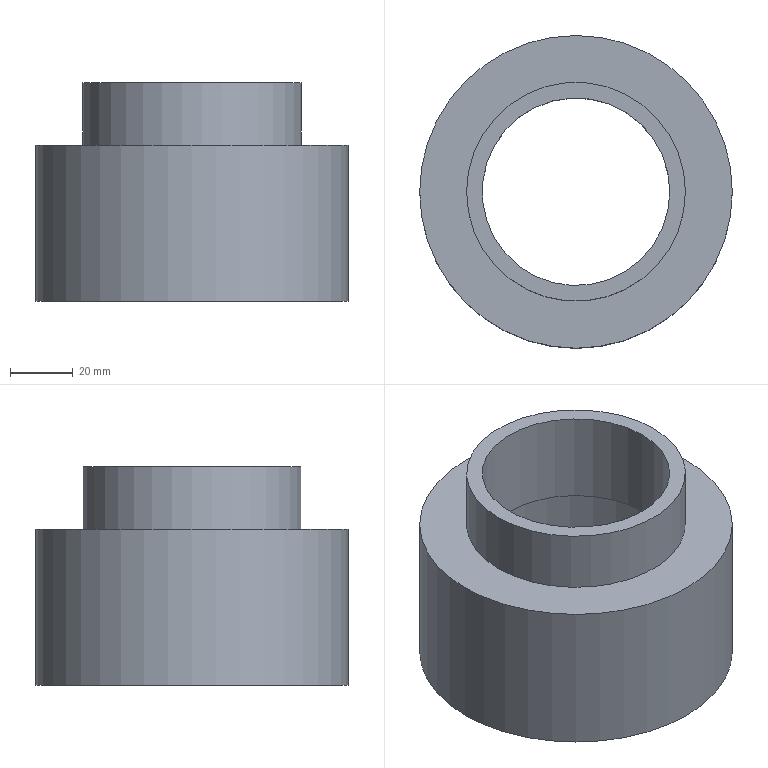Component | NX | CONNECTING_SLEEVE | 1 solid | 8 faces | box 100 x 100 x 70 mm | volume 130376 mm3 | plane 4 | cylinder 4 | commonest cylinder face diameters 100 x1 70 x1 60 x1 90 x1
STEP:
#1=CARTESIAN_POINT('',(0.,0.,0.));
#2=DIRECTION('',(0.,0.,1.));
#3=DIRECTION('',(1.,0.,0.));
#4=AXIS2_PLACEMENT_3D('',#1,#2,#3);
#5=CARTESIAN_POINT('',(35.,0.,-612.5));
#6=VERTEX_POINT('',#5);
#7=CARTESIAN_POINT('',(-0.,0.,-612.5));
#8=DIRECTION('',(0.,0.,1.));
#9=DIRECTION('',(1.,0.,0.));
#10=AXIS2_PLACEMENT_3D('',#7,#8,#9);
#11=CIRCLE('',#10,35.);
#12=CARTESIAN_POINT('',(0.,0.,-612.5));
#13=DIRECTION('',(0.,0.,1.));
#14=DIRECTION('',(1.,0.,0.));
#15=AXIS2_PLACEMENT_3D('',#12,#13,#14);
#16=PLANE('',#15);
#17=CARTESIAN_POINT('',(-0.,-0.));
#18=DIRECTION('',(1.,0.));
#19=AXIS2_PLACEMENT_2D('',#17,#18);
#20=CIRCLE('',#19,35.);
#21=(GEOMETRIC_REPRESENTATION_CONTEXT(2)PARAMETRIC_REPRESENTATION_CONTEXT()REPRESENTATION_CONTEXT('',''));
#22=DEFINITIONAL_REPRESENTATION('',(#20),#21);
#23=PCURVE('',#16,#22);
#24=CARTESIAN_POINT('',(-0.,0.,-612.5));
#25=DIRECTION('',(0.,0.,1.));
#26=DIRECTION('',(1.,0.,0.));
#27=AXIS2_PLACEMENT_3D('',#24,#25,#26);
#28=CYLINDRICAL_SURFACE('',#27,35.);
#29=CARTESIAN_POINT('',(0.,0.));
#30=DIRECTION('',(1.,0.));
#31=VECTOR('',#30,1.);
#32=LINE('',#29,#31);
#33=(GEOMETRIC_REPRESENTATION_CONTEXT(2)PARAMETRIC_REPRESENTATION_CONTEXT()REPRESENTATION_CONTEXT('',''));
#34=DEFINITIONAL_REPRESENTATION('',(#32),#33);
#35=PCURVE('',#28,#34);
#36=SURFACE_CURVE('',#11,(#23,#35),.PCURVE_S1.);
#37=EDGE_CURVE('',#6,#6,#36,.T.);
#38=ORIENTED_EDGE('',*,*,#37,.F.);
#39=EDGE_LOOP('',(#38));
#40=FACE_BOUND('',#39,.T.);
#41=CARTESIAN_POINT('',(50.,0.,-612.5));
#42=VERTEX_POINT('',#41);
#43=CARTESIAN_POINT('',(0.,0.,-612.5));
#44=DIRECTION('',(0.,0.,-1.));
#45=DIRECTION('',(1.,0.,0.));
#46=AXIS2_PLACEMENT_3D('',#43,#44,#45);
#47=CIRCLE('',#46,50.);
#48=CARTESIAN_POINT('',(50.,0.));
#49=CARTESIAN_POINT('',(50.,-86.603));
#50=CARTESIAN_POINT('',(-25.,-43.301));
#51=CARTESIAN_POINT('',(-100.,-0.));
#52=CARTESIAN_POINT('',(-25.,43.301));
#53=CARTESIAN_POINT('',(50.,86.603));
#54=CARTESIAN_POINT('',(50.,0.));
#55=(BOUNDED_CURVE()B_SPLINE_CURVE(2,(#48,#49,#50,#51,#52,#53,#54),.UNSPECIFIED.,.T.,.F.)B_SPLINE_CURVE_WITH_KNOTS((1,2,2,2,2,1),(-2.094,0.,2.094,4.189,6.283,8.378),.UNSPECIFIED.)CURVE()GEOMETRIC_REPRESENTATION_ITEM()RATIONAL_B_SPLINE_CURVE((1.,0.5,1.,0.5,1.,0.5,1.))REPRESENTATION_ITEM(''));
#56=(GEOMETRIC_REPRESENTATION_CONTEXT(2)PARAMETRIC_REPRESENTATION_CONTEXT()REPRESENTATION_CONTEXT('',''));
#57=DEFINITIONAL_REPRESENTATION('',(#55),#56);
#58=PCURVE('',#16,#57);
#59=CARTESIAN_POINT('',(0.,0.,-662.5));
#60=DIRECTION('',(0.,0.,1.));
#61=DIRECTION('',(1.,0.,0.));
#62=AXIS2_PLACEMENT_3D('',#59,#60,#61);
#63=CYLINDRICAL_SURFACE('',#62,50.);
#64=CARTESIAN_POINT('',(6.283,50.));
#65=DIRECTION('',(-1.,0.));
#66=VECTOR('',#65,1.);
#67=LINE('',#64,#66);
#68=(GEOMETRIC_REPRESENTATION_CONTEXT(2)PARAMETRIC_REPRESENTATION_CONTEXT()REPRESENTATION_CONTEXT('',''));
#69=DEFINITIONAL_REPRESENTATION('',(#67),#68);
#70=PCURVE('',#63,#69);
#71=SURFACE_CURVE('',#47,(#58,#70),.PCURVE_S1.);
#72=EDGE_CURVE('',#42,#42,#71,.T.);
#73=ORIENTED_EDGE('',*,*,#72,.F.);
#74=EDGE_LOOP('',(#73));
#75=FACE_BOUND('',#74,.T.);
#76=ADVANCED_FACE('',(#40,#75),#16,.T.);
#77=CARTESIAN_POINT('',(45.,0.,-662.5));
#78=VERTEX_POINT('',#77);
#79=CARTESIAN_POINT('',(-0.,0.,-662.5));
#80=DIRECTION('',(0.,0.,1.));
#81=DIRECTION('',(1.,0.,0.));
#82=AXIS2_PLACEMENT_3D('',#79,#80,#81);
#83=CIRCLE('',#82,45.);
#84=CARTESIAN_POINT('',(0.,0.,-662.5));
#85=DIRECTION('',(0.,0.,-1.));
#86=DIRECTION('',(-1.,0.,0.));
#87=AXIS2_PLACEMENT_3D('',#84,#85,#86);
#88=PLANE('',#87);
#89=CARTESIAN_POINT('',(-45.,-0.));
#90=CARTESIAN_POINT('',(-45.,77.942));
#91=CARTESIAN_POINT('',(22.5,38.971));
#92=CARTESIAN_POINT('',(90.,0.));
#93=CARTESIAN_POINT('',(22.5,-38.971));
#94=CARTESIAN_POINT('',(-45.,-77.942));
#95=CARTESIAN_POINT('',(-45.,-0.));
#96=(BOUNDED_CURVE()B_SPLINE_CURVE(2,(#89,#90,#91,#92,#93,#94,#95),.UNSPECIFIED.,.T.,.F.)B_SPLINE_CURVE_WITH_KNOTS((1,2,2,2,2,1),(-2.094,0.,2.094,4.189,6.283,8.378),.UNSPECIFIED.)CURVE()GEOMETRIC_REPRESENTATION_ITEM()RATIONAL_B_SPLINE_CURVE((1.,0.5,1.,0.5,1.,0.5,1.))REPRESENTATION_ITEM(''));
#97=(GEOMETRIC_REPRESENTATION_CONTEXT(2)PARAMETRIC_REPRESENTATION_CONTEXT()REPRESENTATION_CONTEXT('',''));
#98=DEFINITIONAL_REPRESENTATION('',(#96),#97);
#99=PCURVE('',#88,#98);
#100=CARTESIAN_POINT('',(-0.,0.,-622.5));
#101=DIRECTION('',(0.,0.,-1.));
#102=DIRECTION('',(-1.,0.,0.));
#103=AXIS2_PLACEMENT_3D('',#100,#101,#102);
#104=CYLINDRICAL_SURFACE('',#103,45.);
#105=CARTESIAN_POINT('',(9.425,40.));
#106=DIRECTION('',(-1.,0.));
#107=VECTOR('',#106,1.);
#108=LINE('',#105,#107);
#109=(GEOMETRIC_REPRESENTATION_CONTEXT(2)PARAMETRIC_REPRESENTATION_CONTEXT()REPRESENTATION_CONTEXT('',''));
#110=DEFINITIONAL_REPRESENTATION('',(#108),#109);
#111=PCURVE('',#104,#110);
#112=SURFACE_CURVE('',#83,(#99,#111),.PCURVE_S1.);
#113=EDGE_CURVE('',#78,#78,#112,.T.);
#114=ORIENTED_EDGE('',*,*,#113,.T.);
#115=EDGE_LOOP('',(#114));
#116=FACE_BOUND('',#115,.T.);
#117=CARTESIAN_POINT('',(50.,0.,-662.5));
#118=VERTEX_POINT('',#117);
#119=CARTESIAN_POINT('',(0.,0.,-662.5));
#120=DIRECTION('',(0.,0.,1.));
#121=DIRECTION('',(1.,0.,0.));
#122=AXIS2_PLACEMENT_3D('',#119,#120,#121);
#123=CIRCLE('',#122,50.);
#124=CARTESIAN_POINT('',(-50.,0.));
#125=CARTESIAN_POINT('',(-50.,86.603));
#126=CARTESIAN_POINT('',(25.,43.301));
#127=CARTESIAN_POINT('',(100.,0.));
#128=CARTESIAN_POINT('',(25.,-43.301));
#129=CARTESIAN_POINT('',(-50.,-86.603));
#130=CARTESIAN_POINT('',(-50.,0.));
#131=(BOUNDED_CURVE()B_SPLINE_CURVE(2,(#124,#125,#126,#127,#128,#129,#130),.UNSPECIFIED.,.T.,.F.)B_SPLINE_CURVE_WITH_KNOTS((1,2,2,2,2,1),(-2.094,0.,2.094,4.189,6.283,8.378),.UNSPECIFIED.)CURVE()GEOMETRIC_REPRESENTATION_ITEM()RATIONAL_B_SPLINE_CURVE((1.,0.5,1.,0.5,1.,0.5,1.))REPRESENTATION_ITEM(''));
#132=(GEOMETRIC_REPRESENTATION_CONTEXT(2)PARAMETRIC_REPRESENTATION_CONTEXT()REPRESENTATION_CONTEXT('',''));
#133=DEFINITIONAL_REPRESENTATION('',(#131),#132);
#134=PCURVE('',#88,#133);
#135=CARTESIAN_POINT('',(0.,0.));
#136=DIRECTION('',(1.,0.));
#137=VECTOR('',#136,1.);
#138=LINE('',#135,#137);
#139=(GEOMETRIC_REPRESENTATION_CONTEXT(2)PARAMETRIC_REPRESENTATION_CONTEXT()REPRESENTATION_CONTEXT('',''));
#140=DEFINITIONAL_REPRESENTATION('',(#138),#139);
#141=PCURVE('',#63,#140);
#142=SURFACE_CURVE('',#123,(#134,#141),.PCURVE_S1.);
#143=EDGE_CURVE('',#118,#118,#142,.T.);
#144=ORIENTED_EDGE('',*,*,#143,.F.);
#145=EDGE_LOOP('',(#144));
#146=FACE_BOUND('',#145,.T.);
#147=ADVANCED_FACE('',(#116,#146),#88,.T.);
#148=ORIENTED_EDGE('',*,*,#72,.T.);
#149=CARTESIAN_POINT('',(50.,-0.,-662.5));
#150=CARTESIAN_POINT('',(50.,-0.,-612.5));
#151=B_SPLINE_CURVE_WITH_KNOTS('',1,(#149,#150),.UNSPECIFIED.,.F.,.F.,(2,2),(0.,50.),.PIECEWISE_BEZIER_KNOTS.);
#152=CARTESIAN_POINT('',(0.,0.));
#153=DIRECTION('',(0.,1.));
#154=VECTOR('',#153,1.);
#155=LINE('',#152,#154);
#156=(GEOMETRIC_REPRESENTATION_CONTEXT(2)PARAMETRIC_REPRESENTATION_CONTEXT()REPRESENTATION_CONTEXT('',''));
#157=DEFINITIONAL_REPRESENTATION('',(#155),#156);
#158=PCURVE('',#63,#157);
#159=CARTESIAN_POINT('',(6.283,0.));
#160=DIRECTION('',(0.,1.));
#161=VECTOR('',#160,1.);
#162=LINE('',#159,#161);
#163=(GEOMETRIC_REPRESENTATION_CONTEXT(2)PARAMETRIC_REPRESENTATION_CONTEXT()REPRESENTATION_CONTEXT('',''));
#164=DEFINITIONAL_REPRESENTATION('',(#162),#163);
#165=PCURVE('',#63,#164);
#166=SEAM_CURVE('',#151,(#158,#165),.PCURVE_S1.);
#167=EDGE_CURVE('',#118,#42,#166,.T.);
#168=ORIENTED_EDGE('',*,*,#167,.F.);
#169=ORIENTED_EDGE('',*,*,#143,.T.);
#170=ORIENTED_EDGE('',*,*,#167,.T.);
#171=EDGE_LOOP('',(#148,#168,#169,#170));
#172=FACE_BOUND('',#171,.T.);
#173=ADVANCED_FACE('',(#172),#63,.T.);
#174=CARTESIAN_POINT('',(30.,0.,-592.5));
#175=VERTEX_POINT('',#174);
#176=CARTESIAN_POINT('',(0.,0.,-592.5));
#177=DIRECTION('',(0.,0.,-1.));
#178=DIRECTION('',(1.,0.,0.));
#179=AXIS2_PLACEMENT_3D('',#176,#177,#178);
#180=CIRCLE('',#179,30.);
#181=CARTESIAN_POINT('',(-0.,0.,-592.5));
#182=DIRECTION('',(0.,0.,1.));
#183=DIRECTION('',(1.,0.,0.));
#184=AXIS2_PLACEMENT_3D('',#181,#182,#183);
#185=PLANE('',#184);
#186=CARTESIAN_POINT('',(30.,0.));
#187=CARTESIAN_POINT('',(30.,-51.962));
#188=CARTESIAN_POINT('',(-15.,-25.981));
#189=CARTESIAN_POINT('',(-60.,-0.));
#190=CARTESIAN_POINT('',(-15.,25.981));
#191=CARTESIAN_POINT('',(30.,51.962));
#192=CARTESIAN_POINT('',(30.,0.));
#193=(BOUNDED_CURVE()B_SPLINE_CURVE(2,(#186,#187,#188,#189,#190,#191,#192),.UNSPECIFIED.,.T.,.F.)B_SPLINE_CURVE_WITH_KNOTS((1,2,2,2,2,1),(-2.094,0.,2.094,4.189,6.283,8.378),.UNSPECIFIED.)CURVE()GEOMETRIC_REPRESENTATION_ITEM()RATIONAL_B_SPLINE_CURVE((1.,0.5,1.,0.5,1.,0.5,1.))REPRESENTATION_ITEM(''));
#194=(GEOMETRIC_REPRESENTATION_CONTEXT(2)PARAMETRIC_REPRESENTATION_CONTEXT()REPRESENTATION_CONTEXT('',''));
#195=DEFINITIONAL_REPRESENTATION('',(#193),#194);
#196=PCURVE('',#185,#195);
#197=CARTESIAN_POINT('',(0.,0.,-689.5));
#198=DIRECTION('',(0.,0.,1.));
#199=DIRECTION('',(1.,0.,0.));
#200=AXIS2_PLACEMENT_3D('',#197,#198,#199);
#201=CYLINDRICAL_SURFACE('',#200,30.);
#202=CARTESIAN_POINT('',(6.283,97.));
#203=DIRECTION('',(-1.,0.));
#204=VECTOR('',#203,1.);
#205=LINE('',#202,#204);
#206=(GEOMETRIC_REPRESENTATION_CONTEXT(2)PARAMETRIC_REPRESENTATION_CONTEXT()REPRESENTATION_CONTEXT('',''));
#207=DEFINITIONAL_REPRESENTATION('',(#205),#206);
#208=PCURVE('',#201,#207);
#209=SURFACE_CURVE('',#180,(#196,#208),.PCURVE_S1.);
#210=EDGE_CURVE('',#175,#175,#209,.T.);
#211=ORIENTED_EDGE('',*,*,#210,.T.);
#212=EDGE_LOOP('',(#211));
#213=FACE_BOUND('',#212,.T.);
#214=CARTESIAN_POINT('',(35.,0.,-592.5));
#215=VERTEX_POINT('',#214);
#216=CARTESIAN_POINT('',(-0.,0.,-592.5));
#217=DIRECTION('',(0.,0.,1.));
#218=DIRECTION('',(1.,0.,0.));
#219=AXIS2_PLACEMENT_3D('',#216,#217,#218);
#220=CIRCLE('',#219,35.);
#221=CARTESIAN_POINT('',(0.,0.));
#222=DIRECTION('',(1.,0.));
#223=AXIS2_PLACEMENT_2D('',#221,#222);
#224=CIRCLE('',#223,35.);
#225=(GEOMETRIC_REPRESENTATION_CONTEXT(2)PARAMETRIC_REPRESENTATION_CONTEXT()REPRESENTATION_CONTEXT('',''));
#226=DEFINITIONAL_REPRESENTATION('',(#224),#225);
#227=PCURVE('',#185,#226);
#228=CARTESIAN_POINT('',(0.,20.));
#229=DIRECTION('',(1.,0.));
#230=VECTOR('',#229,1.);
#231=LINE('',#228,#230);
#232=(GEOMETRIC_REPRESENTATION_CONTEXT(2)PARAMETRIC_REPRESENTATION_CONTEXT()REPRESENTATION_CONTEXT('',''));
#233=DEFINITIONAL_REPRESENTATION('',(#231),#232);
#234=PCURVE('',#28,#233);
#235=SURFACE_CURVE('',#220,(#227,#234),.PCURVE_S1.);
#236=EDGE_CURVE('',#215,#215,#235,.T.);
#237=ORIENTED_EDGE('',*,*,#236,.T.);
#238=EDGE_LOOP('',(#237));
#239=FACE_BOUND('',#238,.T.);
#240=ADVANCED_FACE('',(#213,#239),#185,.T.);
#241=ORIENTED_EDGE('',*,*,#236,.F.);
#242=CARTESIAN_POINT('',(35.,-0.,-612.5));
#243=CARTESIAN_POINT('',(35.,-0.,-592.5));
#244=B_SPLINE_CURVE_WITH_KNOTS('',1,(#242,#243),.UNSPECIFIED.,.F.,.F.,(2,2),(0.,20.),.PIECEWISE_BEZIER_KNOTS.);
#245=CARTESIAN_POINT('',(0.,0.));
#246=DIRECTION('',(0.,1.));
#247=VECTOR('',#246,1.);
#248=LINE('',#245,#247);
#249=(GEOMETRIC_REPRESENTATION_CONTEXT(2)PARAMETRIC_REPRESENTATION_CONTEXT()REPRESENTATION_CONTEXT('',''));
#250=DEFINITIONAL_REPRESENTATION('',(#248),#249);
#251=PCURVE('',#28,#250);
#252=CARTESIAN_POINT('',(6.283,0.));
#253=DIRECTION('',(0.,1.));
#254=VECTOR('',#253,1.);
#255=LINE('',#252,#254);
#256=(GEOMETRIC_REPRESENTATION_CONTEXT(2)PARAMETRIC_REPRESENTATION_CONTEXT()REPRESENTATION_CONTEXT('',''));
#257=DEFINITIONAL_REPRESENTATION('',(#255),#256);
#258=PCURVE('',#28,#257);
#259=SEAM_CURVE('',#244,(#251,#258),.PCURVE_S1.);
#260=EDGE_CURVE('',#6,#215,#259,.T.);
#261=ORIENTED_EDGE('',*,*,#260,.F.);
#262=ORIENTED_EDGE('',*,*,#37,.T.);
#263=ORIENTED_EDGE('',*,*,#260,.T.);
#264=EDGE_LOOP('',(#241,#261,#262,#263));
#265=FACE_BOUND('',#264,.T.);
#266=ADVANCED_FACE('',(#265),#28,.T.);
#267=CARTESIAN_POINT('',(30.,0.,-622.5));
#268=VERTEX_POINT('',#267);
#269=CARTESIAN_POINT('',(0.,0.,-622.5));
#270=DIRECTION('',(0.,0.,1.));
#271=DIRECTION('',(1.,0.,0.));
#272=AXIS2_PLACEMENT_3D('',#269,#270,#271);
#273=CIRCLE('',#272,30.);
#274=CARTESIAN_POINT('',(0.,67.));
#275=DIRECTION('',(1.,0.));
#276=VECTOR('',#275,1.);
#277=LINE('',#274,#276);
#278=(GEOMETRIC_REPRESENTATION_CONTEXT(2)PARAMETRIC_REPRESENTATION_CONTEXT()REPRESENTATION_CONTEXT('',''));
#279=DEFINITIONAL_REPRESENTATION('',(#277),#278);
#280=PCURVE('',#201,#279);
#281=CARTESIAN_POINT('',(-0.,0.,-622.5));
#282=DIRECTION('',(0.,0.,1.));
#283=DIRECTION('',(1.,0.,0.));
#284=AXIS2_PLACEMENT_3D('',#281,#282,#283);
#285=PLANE('',#284);
#286=CARTESIAN_POINT('',(0.,0.));
#287=DIRECTION('',(1.,0.));
#288=AXIS2_PLACEMENT_2D('',#286,#287);
#289=CIRCLE('',#288,30.);
#290=(GEOMETRIC_REPRESENTATION_CONTEXT(2)PARAMETRIC_REPRESENTATION_CONTEXT()REPRESENTATION_CONTEXT('',''));
#291=DEFINITIONAL_REPRESENTATION('',(#289),#290);
#292=PCURVE('',#285,#291);
#293=SURFACE_CURVE('',#273,(#280,#292),.PCURVE_S1.);
#294=EDGE_CURVE('',#268,#268,#293,.T.);
#295=ORIENTED_EDGE('',*,*,#294,.T.);
#296=CARTESIAN_POINT('',(30.,0.,-622.5));
#297=CARTESIAN_POINT('',(30.,0.,-592.5));
#298=B_SPLINE_CURVE_WITH_KNOTS('',1,(#296,#297),.UNSPECIFIED.,.F.,.F.,(2,2),(67.,97.),.PIECEWISE_BEZIER_KNOTS.);
#299=CARTESIAN_POINT('',(6.283,0.));
#300=DIRECTION('',(0.,1.));
#301=VECTOR('',#300,1.);
#302=LINE('',#299,#301);
#303=(GEOMETRIC_REPRESENTATION_CONTEXT(2)PARAMETRIC_REPRESENTATION_CONTEXT()REPRESENTATION_CONTEXT('',''));
#304=DEFINITIONAL_REPRESENTATION('',(#302),#303);
#305=PCURVE('',#201,#304);
#306=CARTESIAN_POINT('',(0.,0.));
#307=DIRECTION('',(0.,1.));
#308=VECTOR('',#307,1.);
#309=LINE('',#306,#308);
#310=(GEOMETRIC_REPRESENTATION_CONTEXT(2)PARAMETRIC_REPRESENTATION_CONTEXT()REPRESENTATION_CONTEXT('',''));
#311=DEFINITIONAL_REPRESENTATION('',(#309),#310);
#312=PCURVE('',#201,#311);
#313=SEAM_CURVE('',#298,(#305,#312),.PCURVE_S1.);
#314=EDGE_CURVE('',#268,#175,#313,.T.);
#315=ORIENTED_EDGE('',*,*,#314,.T.);
#316=ORIENTED_EDGE('',*,*,#210,.T.);
#317=ORIENTED_EDGE('',*,*,#314,.F.);
#318=EDGE_LOOP('',(#295,#315,#316,#317));
#319=FACE_BOUND('',#318,.F.);
#320=ADVANCED_FACE('',(#319),#201,.F.);
#321=CARTESIAN_POINT('',(45.,0.,-622.5));
#322=VERTEX_POINT('',#321);
#323=CARTESIAN_POINT('',(-0.,0.,-622.5));
#324=DIRECTION('',(0.,0.,-1.));
#325=DIRECTION('',(1.,0.,0.));
#326=AXIS2_PLACEMENT_3D('',#323,#324,#325);
#327=CIRCLE('',#326,45.);
#328=CARTESIAN_POINT('',(3.142,0.));
#329=DIRECTION('',(1.,0.));
#330=VECTOR('',#329,1.);
#331=LINE('',#328,#330);
#332=(GEOMETRIC_REPRESENTATION_CONTEXT(2)PARAMETRIC_REPRESENTATION_CONTEXT()REPRESENTATION_CONTEXT('',''));
#333=DEFINITIONAL_REPRESENTATION('',(#331),#332);
#334=PCURVE('',#104,#333);
#335=CARTESIAN_POINT('',(45.,0.));
#336=CARTESIAN_POINT('',(45.,-77.942));
#337=CARTESIAN_POINT('',(-22.5,-38.971));
#338=CARTESIAN_POINT('',(-90.,-0.));
#339=CARTESIAN_POINT('',(-22.5,38.971));
#340=CARTESIAN_POINT('',(45.,77.942));
#341=CARTESIAN_POINT('',(45.,0.));
#342=(BOUNDED_CURVE()B_SPLINE_CURVE(2,(#335,#336,#337,#338,#339,#340,#341),.UNSPECIFIED.,.T.,.F.)B_SPLINE_CURVE_WITH_KNOTS((1,2,2,2,2,1),(-2.094,0.,2.094,4.189,6.283,8.378),.UNSPECIFIED.)CURVE()GEOMETRIC_REPRESENTATION_ITEM()RATIONAL_B_SPLINE_CURVE((1.,0.5,1.,0.5,1.,0.5,1.))REPRESENTATION_ITEM(''));
#343=(GEOMETRIC_REPRESENTATION_CONTEXT(2)PARAMETRIC_REPRESENTATION_CONTEXT()REPRESENTATION_CONTEXT('',''));
#344=DEFINITIONAL_REPRESENTATION('',(#342),#343);
#345=PCURVE('',#285,#344);
#346=SURFACE_CURVE('',#327,(#334,#345),.PCURVE_S1.);
#347=EDGE_CURVE('',#322,#322,#346,.T.);
#348=ORIENTED_EDGE('',*,*,#347,.T.);
#349=CARTESIAN_POINT('',(45.,0.,-622.5));
#350=CARTESIAN_POINT('',(45.,0.,-662.5));
#351=B_SPLINE_CURVE_WITH_KNOTS('',1,(#349,#350),.UNSPECIFIED.,.F.,.F.,(2,2),(0.,40.),.PIECEWISE_BEZIER_KNOTS.);
#352=CARTESIAN_POINT('',(9.425,0.));
#353=DIRECTION('',(0.,1.));
#354=VECTOR('',#353,1.);
#355=LINE('',#352,#354);
#356=(GEOMETRIC_REPRESENTATION_CONTEXT(2)PARAMETRIC_REPRESENTATION_CONTEXT()REPRESENTATION_CONTEXT('',''));
#357=DEFINITIONAL_REPRESENTATION('',(#355),#356);
#358=PCURVE('',#104,#357);
#359=CARTESIAN_POINT('',(3.142,0.));
#360=DIRECTION('',(0.,1.));
#361=VECTOR('',#360,1.);
#362=LINE('',#359,#361);
#363=(GEOMETRIC_REPRESENTATION_CONTEXT(2)PARAMETRIC_REPRESENTATION_CONTEXT()REPRESENTATION_CONTEXT('',''));
#364=DEFINITIONAL_REPRESENTATION('',(#362),#363);
#365=PCURVE('',#104,#364);
#366=SEAM_CURVE('',#351,(#358,#365),.PCURVE_S1.);
#367=EDGE_CURVE('',#322,#78,#366,.T.);
#368=ORIENTED_EDGE('',*,*,#367,.T.);
#369=ORIENTED_EDGE('',*,*,#113,.T.);
#370=ORIENTED_EDGE('',*,*,#367,.F.);
#371=EDGE_LOOP('',(#348,#368,#369,#370));
#372=FACE_BOUND('',#371,.F.);
#373=ADVANCED_FACE('',(#372),#104,.F.);
#374=ORIENTED_EDGE('',*,*,#294,.T.);
#375=EDGE_LOOP('',(#374));
#376=FACE_BOUND('',#375,.T.);
#377=ORIENTED_EDGE('',*,*,#347,.T.);
#378=EDGE_LOOP('',(#377));
#379=FACE_BOUND('',#378,.T.);
#380=ADVANCED_FACE('',(#376,#379),#285,.F.);
#381=CLOSED_SHELL('',(#76,#147,#173,#240,#266,#320,#373,#380));
#382=MANIFOLD_SOLID_BREP('',#381);
#383=(LENGTH_UNIT()NAMED_UNIT(*)SI_UNIT(.MILLI.,.METRE.));
#384=UNCERTAINTY_MEASURE_WITH_UNIT(LENGTH_MEASURE(0.00001),#383,'','');
#385=(NAMED_UNIT(*)PLANE_ANGLE_UNIT()SI_UNIT($,.RADIAN.));
#386=(NAMED_UNIT(*)SI_UNIT($,.STERADIAN.)SOLID_ANGLE_UNIT());
#387=(GEOMETRIC_REPRESENTATION_CONTEXT(3)GLOBAL_UNCERTAINTY_ASSIGNED_CONTEXT((#384))GLOBAL_UNIT_ASSIGNED_CONTEXT((#383,#385,#386))REPRESENTATION_CONTEXT('',''));
#388=ADVANCED_BREP_SHAPE_REPRESENTATION('',(#4,#382),#387);